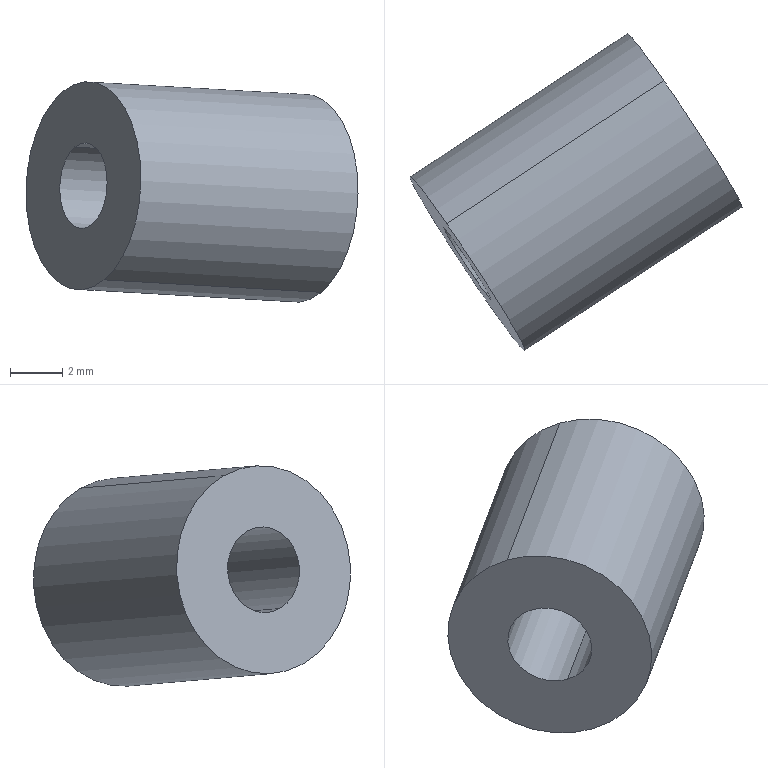Component | SolidWorks | DoorGasket-1 | 1 solid | 6 faces | box 12.75 x 12.18 x 8.47 mm | volume 417 mm3 | cylinder 4 | plane 2 | commonest cylinder face diameters 3.3 x2 8 x2
build123d program:
from build123d import *

# Parameters (mm, degrees)
SKETCH1_R           = 4
BOSS_EXTRUDE1_DEPTH = 10


with BuildPart() as part:
    # Sketch1 → Boss-Extrude1 (new body)
    with BuildSketch(Plane.XY):
        Circle(SKETCH1_R)
    extrude(amount=BOSS_EXTRUDE1_DEPTH)

    # Sketch2 → M4 Tapped Hole1 (revolve, cut)
    with BuildSketch(Plane(origin=(0, 0, 10), x_dir=(0, -1, 0), z_dir=(1, 0, 0))):
        Polygon((0, 0), (0, 11.091), (1.65, 10.1), (1.65, 0), align=None)
    revolve(axis=Axis((0, 0, 16.35), (0, 0, -1)), mode=Mode.SUBTRACT)


solid = part.part

# Placed as in the assembly
solid = solid.moved(Location((-259.235, -27.327, 680.526), (85.021, -56.519, -145.587)))
STEP:
#1=COLOUR_RGB('',0.7922,0.8196,0.9333);
#2=FILL_AREA_STYLE_COLOUR('',#1);
#3=FILL_AREA_STYLE('',(#2));
#4=SURFACE_STYLE_FILL_AREA(#3);
#5=SURFACE_SIDE_STYLE('',(#4));
#6=SURFACE_STYLE_USAGE(.BOTH.,#5);
#7=PRESENTATION_STYLE_ASSIGNMENT((#6));
#8=CARTESIAN_POINT('',(-10.522,-1.317,26.753));
#9=VERTEX_POINT('',#8);
#10=CARTESIAN_POINT('',(-10.547,-1.268,26.87));
#11=VERTEX_POINT('',#10);
#12=CARTESIAN_POINT('',(-10.534,-1.292,26.811));
#13=DIRECTION('',(0.8341,0.5496,-0.04788));
#14=DIRECTION('',(-0.1983,0.3796,0.9036));
#15=AXIS2_PLACEMENT_3D('',#12,#13,#14);
#16=CIRCLE('',#15,0.06496);
#17=EDGE_CURVE('',#9,#11,#16,.T.);
#18=ORIENTED_EDGE('',*,*,#17,.F.);
#19=CARTESIAN_POINT('',(-10.193,-1.101,26.734));
#20=VERTEX_POINT('',#19);
#21=CARTESIAN_POINT('',(-10.193,-1.101,26.734));
#22=DIRECTION('',(0.8341,0.5496,-0.04788));
#23=VECTOR('',#22,39.37);
#24=LINE('',#21,#23);
#25=EDGE_CURVE('',#9,#20,#24,.T.);
#26=ORIENTED_EDGE('',*,*,#25,.T.);
#27=CARTESIAN_POINT('',(-10.219,-1.051,26.851));
#28=VERTEX_POINT('',#27);
#29=CARTESIAN_POINT('',(-10.206,-1.076,26.792));
#30=DIRECTION('',(0.8341,0.5496,-0.04788));
#31=DIRECTION('',(-0.1983,0.3796,0.9036));
#32=AXIS2_PLACEMENT_3D('',#29,#30,#31);
#33=CIRCLE('',#32,0.06496);
#34=EDGE_CURVE('',#20,#28,#33,.T.);
#35=ORIENTED_EDGE('',*,*,#34,.T.);
#36=CARTESIAN_POINT('',(-10.219,-1.051,26.851));
#37=DIRECTION('',(0.8341,0.5496,-0.04788));
#38=VECTOR('',#37,39.37);
#39=LINE('',#36,#38);
#40=EDGE_CURVE('',#11,#28,#39,.T.);
#41=ORIENTED_EDGE('',*,*,#40,.F.);
#42=EDGE_LOOP('',(#18,#26,#35,#41));
#43=FACE_OUTER_BOUND('',#42,.T.);
#44=CARTESIAN_POINT('',(-10.206,-1.076,26.792));
#45=DIRECTION('',(0.8341,0.5496,-0.04788));
#46=DIRECTION('',(-0.1983,0.3796,0.9036));
#47=AXIS2_PLACEMENT_3D('',#44,#45,#46);
#48=CYLINDRICAL_SURFACE('',#47,0.06496);
#49=ADVANCED_FACE('',(#43),#48,.F.);
#50=CARTESIAN_POINT('',(-10.237,-1.016,26.935));
#51=VERTEX_POINT('',#50);
#52=CARTESIAN_POINT('',(-10.175,-1.136,26.65));
#53=VERTEX_POINT('',#52);
#54=CARTESIAN_POINT('',(-10.206,-1.076,26.792));
#55=DIRECTION('',(0.8341,0.5496,-0.04788));
#56=DIRECTION('',(-0.1983,0.3796,0.9036));
#57=AXIS2_PLACEMENT_3D('',#54,#55,#56);
#58=CIRCLE('',#57,0.1575);
#59=EDGE_CURVE('',#51,#53,#58,.T.);
#60=ORIENTED_EDGE('',*,*,#59,.F.);
#61=CARTESIAN_POINT('',(-10.566,-1.232,26.954));
#62=VERTEX_POINT('',#61);
#63=CARTESIAN_POINT('',(-10.237,-1.016,26.935));
#64=DIRECTION('',(-0.8341,-0.5496,0.04788));
#65=VECTOR('',#64,39.37);
#66=LINE('',#63,#65);
#67=EDGE_CURVE('',#51,#62,#66,.T.);
#68=ORIENTED_EDGE('',*,*,#67,.T.);
#69=CARTESIAN_POINT('',(-10.503,-1.352,26.669));
#70=VERTEX_POINT('',#69);
#71=CARTESIAN_POINT('',(-10.534,-1.292,26.811));
#72=DIRECTION('',(0.8341,0.5496,-0.04788));
#73=DIRECTION('',(-0.1983,0.3796,0.9036));
#74=AXIS2_PLACEMENT_3D('',#71,#72,#73);
#75=CIRCLE('',#74,0.1575);
#76=EDGE_CURVE('',#62,#70,#75,.T.);
#77=ORIENTED_EDGE('',*,*,#76,.T.);
#78=CARTESIAN_POINT('',(-10.175,-1.136,26.65));
#79=DIRECTION('',(-0.8341,-0.5496,0.04788));
#80=VECTOR('',#79,39.37);
#81=LINE('',#78,#80);
#82=EDGE_CURVE('',#53,#70,#81,.T.);
#83=ORIENTED_EDGE('',*,*,#82,.F.);
#84=EDGE_LOOP('',(#60,#68,#77,#83));
#85=FACE_OUTER_BOUND('',#84,.T.);
#86=CARTESIAN_POINT('',(-10.206,-1.076,26.792));
#87=DIRECTION('',(-0.8341,-0.5496,0.04788));
#88=DIRECTION('',(0.1983,-0.3796,-0.9036));
#89=AXIS2_PLACEMENT_3D('',#86,#87,#88);
#90=CYLINDRICAL_SURFACE('',#89,0.1575);
#91=ADVANCED_FACE('',(#85),#90,.T.);
#92=ORIENTED_EDGE('',*,*,#67,.F.);
#93=CARTESIAN_POINT('',(-10.206,-1.076,26.792));
#94=DIRECTION('',(0.8341,0.5496,-0.04788));
#95=DIRECTION('',(-0.1983,0.3796,0.9036));
#96=AXIS2_PLACEMENT_3D('',#93,#94,#95);
#97=CIRCLE('',#96,0.1575);
#98=EDGE_CURVE('',#53,#51,#97,.T.);
#99=ORIENTED_EDGE('',*,*,#98,.F.);
#100=ORIENTED_EDGE('',*,*,#82,.T.);
#101=CARTESIAN_POINT('',(-10.534,-1.292,26.811));
#102=DIRECTION('',(0.8341,0.5496,-0.04788));
#103=DIRECTION('',(-0.1983,0.3796,0.9036));
#104=AXIS2_PLACEMENT_3D('',#101,#102,#103);
#105=CIRCLE('',#104,0.1575);
#106=EDGE_CURVE('',#70,#62,#105,.T.);
#107=ORIENTED_EDGE('',*,*,#106,.T.);
#108=EDGE_LOOP('',(#92,#99,#100,#107));
#109=FACE_OUTER_BOUND('',#108,.T.);
#110=CARTESIAN_POINT('',(-10.206,-1.076,26.792));
#111=DIRECTION('',(-0.8341,-0.5496,0.04788));
#112=DIRECTION('',(0.1983,-0.3796,-0.9036));
#113=AXIS2_PLACEMENT_3D('',#110,#111,#112);
#114=CYLINDRICAL_SURFACE('',#113,0.1575);
#115=ADVANCED_FACE('',(#109),#114,.T.);
#116=CARTESIAN_POINT('',(-10.206,-1.076,26.792));
#117=DIRECTION('',(0.8341,0.5496,-0.04788));
#118=DIRECTION('',(-0.1983,0.3796,0.9036));
#119=AXIS2_PLACEMENT_3D('',#116,#117,#118);
#120=CIRCLE('',#119,0.06496);
#121=EDGE_CURVE('',#28,#20,#120,.T.);
#122=ORIENTED_EDGE('',*,*,#121,.F.);
#123=ORIENTED_EDGE('',*,*,#34,.F.);
#124=EDGE_LOOP('',(#122,#123));
#125=FACE_BOUND('',#124,.T.);
#126=ORIENTED_EDGE('',*,*,#98,.T.);
#127=ORIENTED_EDGE('',*,*,#59,.T.);
#128=EDGE_LOOP('',(#126,#127));
#129=FACE_OUTER_BOUND('',#128,.T.);
#130=CARTESIAN_POINT('',(-10.206,-1.076,26.792));
#131=DIRECTION('',(0.8341,0.5496,-0.04788));
#132=DIRECTION('',(-0.1983,0.3796,0.9036));
#133=AXIS2_PLACEMENT_3D('',#130,#131,#132);
#134=PLANE('',#133);
#135=ADVANCED_FACE('',(#125,#129),#134,.T.);
#136=CARTESIAN_POINT('',(-10.534,-1.292,26.811));
#137=DIRECTION('',(0.8341,0.5496,-0.04788));
#138=DIRECTION('',(-0.1983,0.3796,0.9036));
#139=AXIS2_PLACEMENT_3D('',#136,#137,#138);
#140=CIRCLE('',#139,0.06496);
#141=EDGE_CURVE('',#11,#9,#140,.T.);
#142=ORIENTED_EDGE('',*,*,#141,.T.);
#143=ORIENTED_EDGE('',*,*,#17,.T.);
#144=EDGE_LOOP('',(#142,#143));
#145=FACE_BOUND('',#144,.T.);
#146=ORIENTED_EDGE('',*,*,#106,.F.);
#147=ORIENTED_EDGE('',*,*,#76,.F.);
#148=EDGE_LOOP('',(#146,#147));
#149=FACE_OUTER_BOUND('',#148,.T.);
#150=CARTESIAN_POINT('',(-10.534,-1.292,26.811));
#151=DIRECTION('',(0.8341,0.5496,-0.04788));
#152=DIRECTION('',(-0.1983,0.3796,0.9036));
#153=AXIS2_PLACEMENT_3D('',#150,#151,#152);
#154=PLANE('',#153);
#155=ADVANCED_FACE('',(#145,#149),#154,.F.);
#156=ORIENTED_EDGE('',*,*,#25,.F.);
#157=ORIENTED_EDGE('',*,*,#141,.F.);
#158=ORIENTED_EDGE('',*,*,#40,.T.);
#159=ORIENTED_EDGE('',*,*,#121,.T.);
#160=EDGE_LOOP('',(#156,#157,#158,#159));
#161=FACE_OUTER_BOUND('',#160,.T.);
#162=CARTESIAN_POINT('',(-10.206,-1.076,26.792));
#163=DIRECTION('',(0.8341,0.5496,-0.04788));
#164=DIRECTION('',(-0.1983,0.3796,0.9036));
#165=AXIS2_PLACEMENT_3D('',#162,#163,#164);
#166=CYLINDRICAL_SURFACE('',#165,0.06496);
#167=ADVANCED_FACE('',(#161),#166,.F.);
#168=CLOSED_SHELL('',(#49,#91,#115,#135,#155,#167));
#169=MANIFOLD_SOLID_BREP('',#168);
#170=STYLED_ITEM('',(#7),#169);
#171=(LENGTH_UNIT()NAMED_UNIT(*)SI_UNIT($,.METRE.));
#172=LENGTH_MEASURE_WITH_UNIT(LENGTH_MEASURE(0.0254),#171);
#173=DIMENSIONAL_EXPONENTS(1.,0.,0.,0.,0.,0.,0.);
#174=(CONVERSION_BASED_UNIT('',#172)LENGTH_UNIT()NAMED_UNIT(#173));
#175=UNCERTAINTY_MEASURE_WITH_UNIT(LENGTH_MEASURE(0.00001),#174,'','');
#176=(NAMED_UNIT(*)PLANE_ANGLE_UNIT()SI_UNIT($,.RADIAN.));
#177=(NAMED_UNIT(*)SI_UNIT($,.STERADIAN.)SOLID_ANGLE_UNIT());
#178=(GEOMETRIC_REPRESENTATION_CONTEXT(3)GLOBAL_UNCERTAINTY_ASSIGNED_CONTEXT((#175))GLOBAL_UNIT_ASSIGNED_CONTEXT((#174,#176,#177))REPRESENTATION_CONTEXT('',''));
#179=MECHANICAL_DESIGN_GEOMETRIC_PRESENTATION_REPRESENTATION('',(#170),#178);
#180=PRESENTATION_LAYER_ASSIGNMENT('','',(#170));
#181=CARTESIAN_POINT('',(0.,0.,0.));
#182=DIRECTION('',(0.,0.,1.));
#183=DIRECTION('',(1.,0.,0.));
#184=AXIS2_PLACEMENT_3D('',#181,#182,#183);
#185=(LENGTH_UNIT()NAMED_UNIT(*)SI_UNIT($,.METRE.));
#186=LENGTH_MEASURE_WITH_UNIT(LENGTH_MEASURE(0.0254),#185);
#187=DIMENSIONAL_EXPONENTS(1.,0.,0.,0.,0.,0.,0.);
#188=(CONVERSION_BASED_UNIT('',#186)LENGTH_UNIT()NAMED_UNIT(#187));
#189=UNCERTAINTY_MEASURE_WITH_UNIT(LENGTH_MEASURE(0.00001),#188,'','');
#190=(NAMED_UNIT(*)PLANE_ANGLE_UNIT()SI_UNIT($,.RADIAN.));
#191=(NAMED_UNIT(*)SI_UNIT($,.STERADIAN.)SOLID_ANGLE_UNIT());
#192=(GEOMETRIC_REPRESENTATION_CONTEXT(3)GLOBAL_UNCERTAINTY_ASSIGNED_CONTEXT((#189))GLOBAL_UNIT_ASSIGNED_CONTEXT((#188,#190,#191))REPRESENTATION_CONTEXT('',''));
#193=ADVANCED_BREP_SHAPE_REPRESENTATION('',(#169,#184),#192);